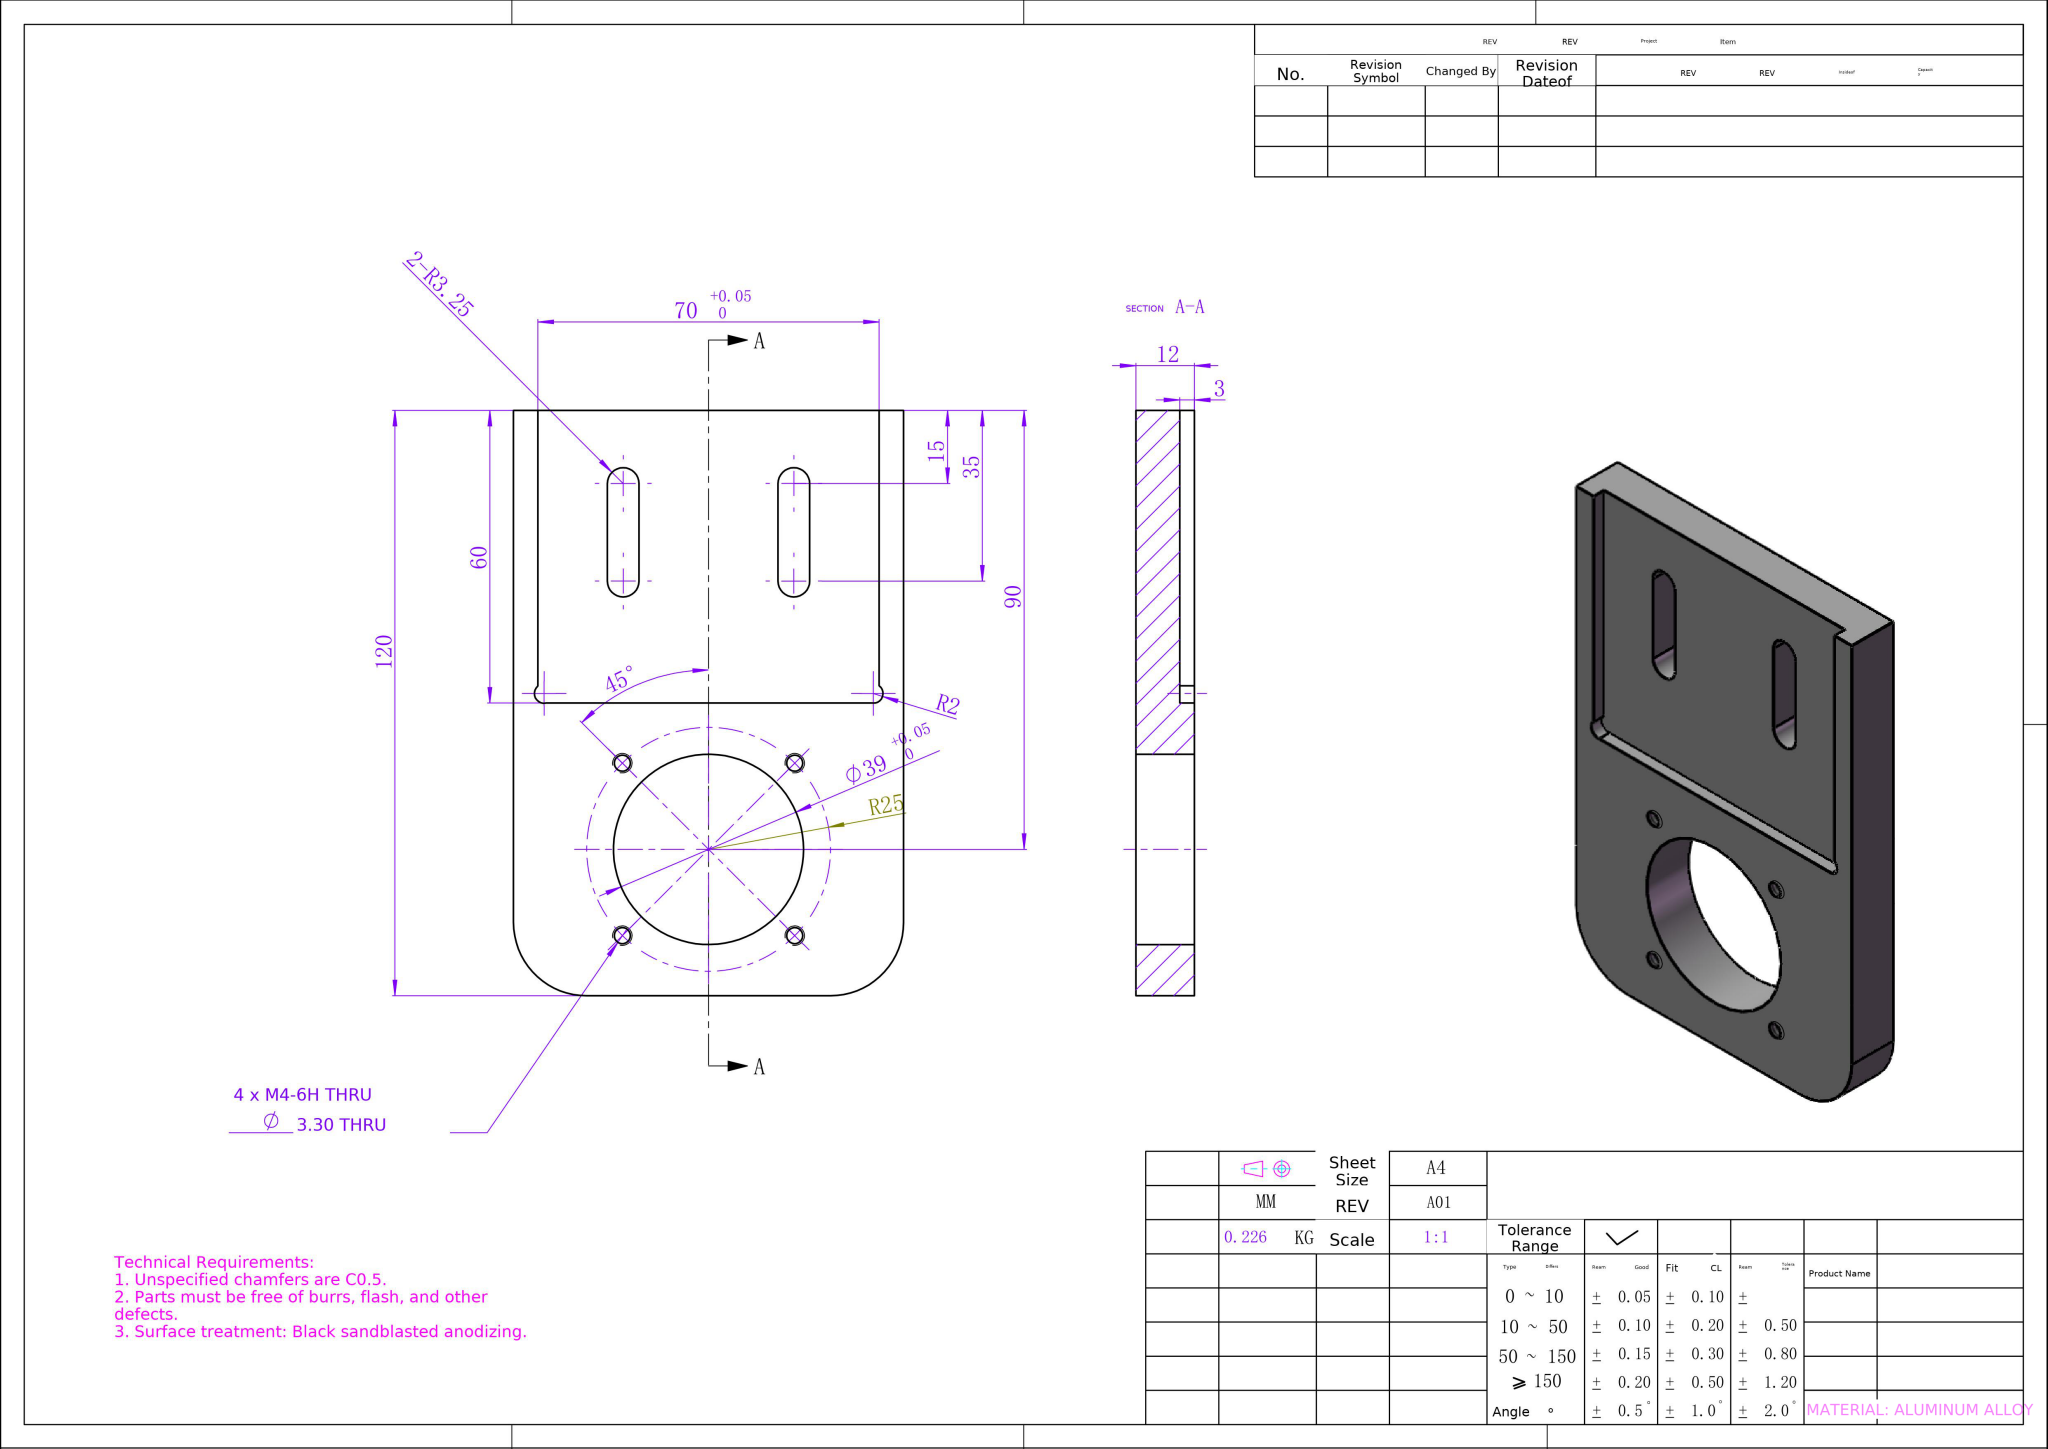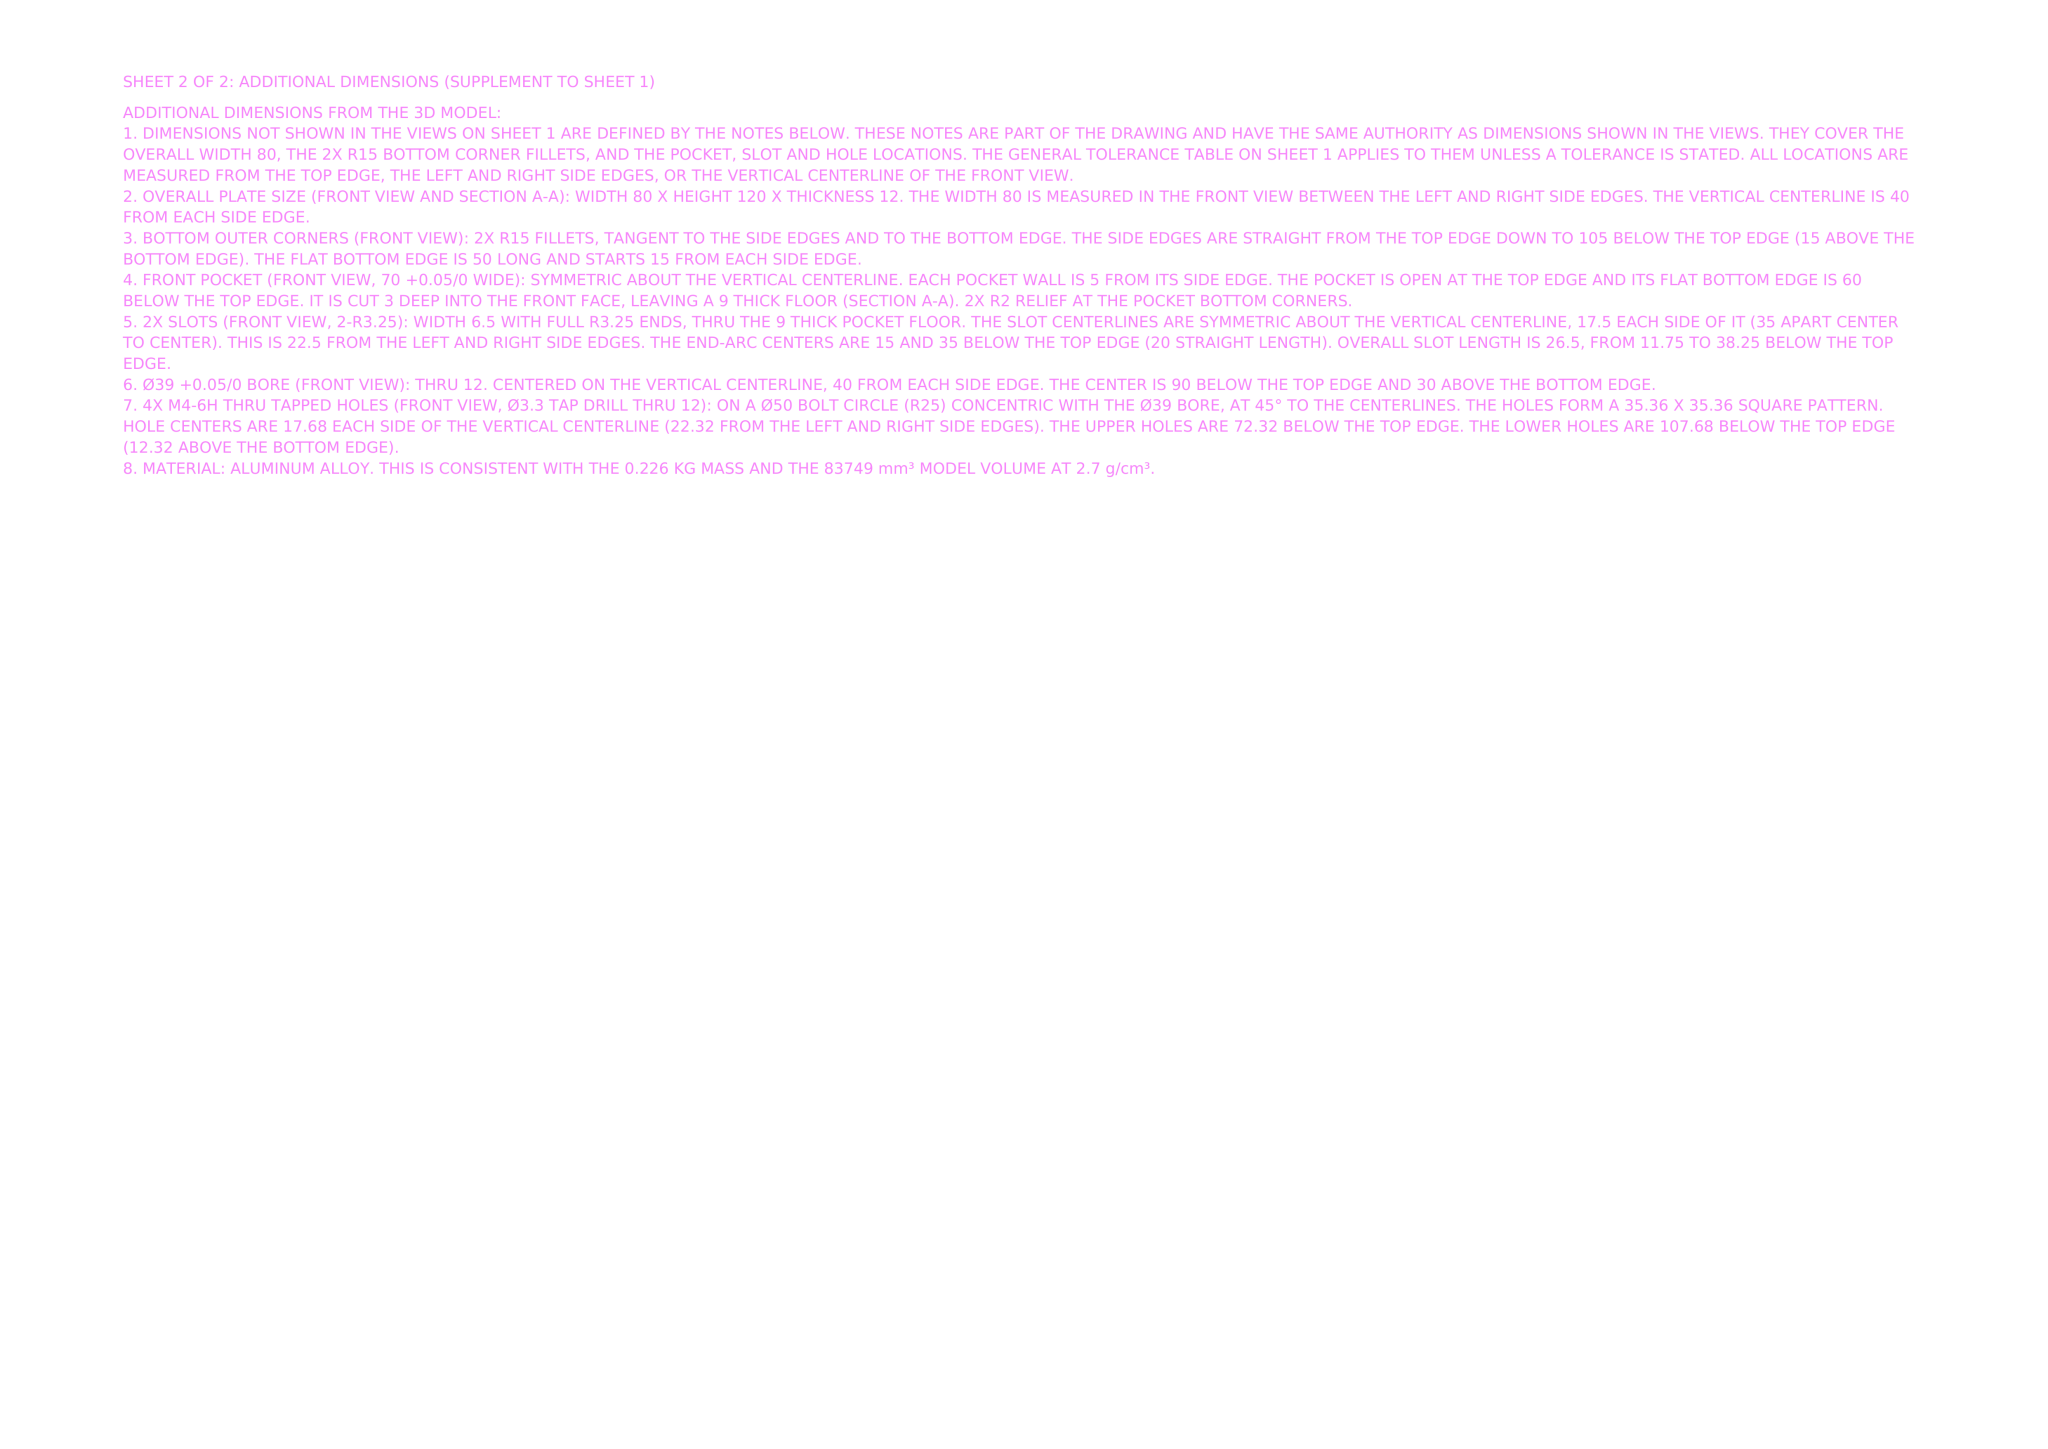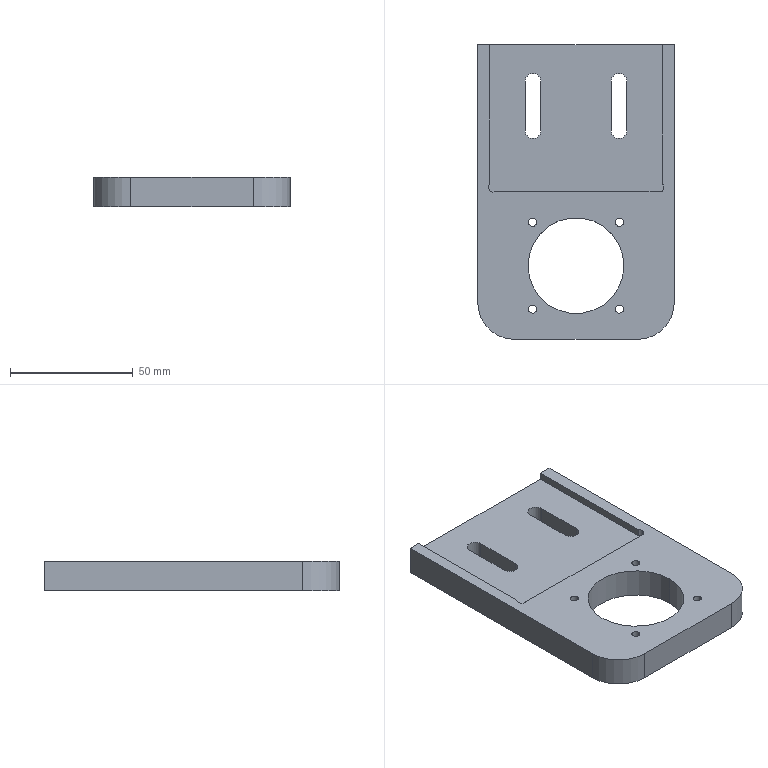Part | NX | mm | 1 solid | 33 faces | box 80 x 120 x 12 mm | volume 83749 mm3 | cylinder 19 | plane 14 | commonest cylinder face diameters 3.3 x8 6.5 x4 4 x3 39 x2 30 x2